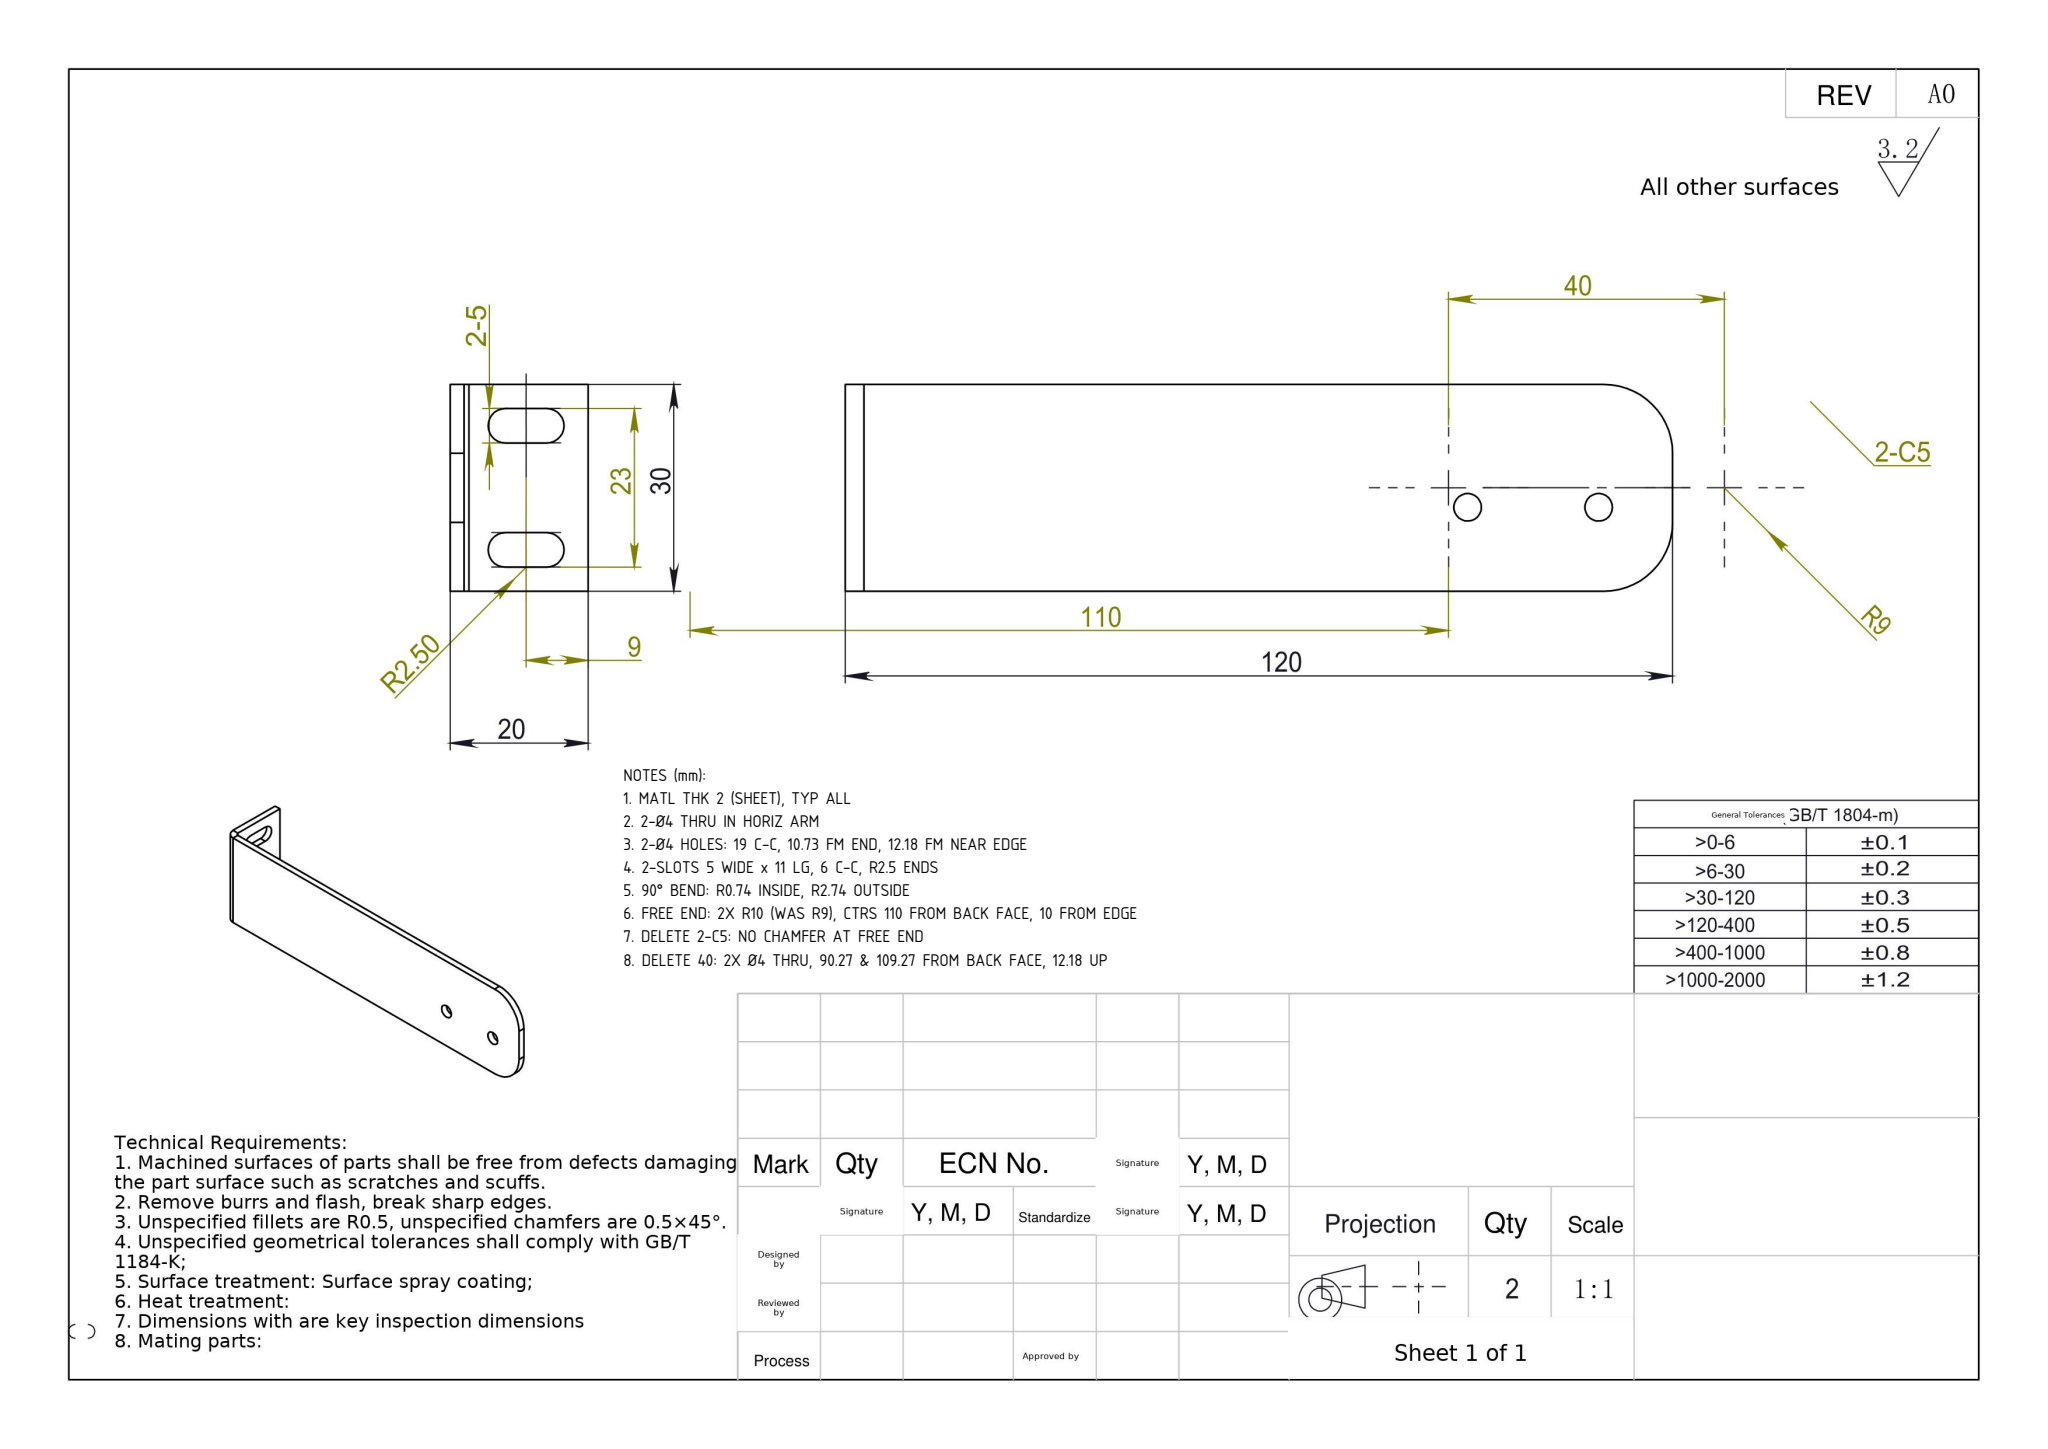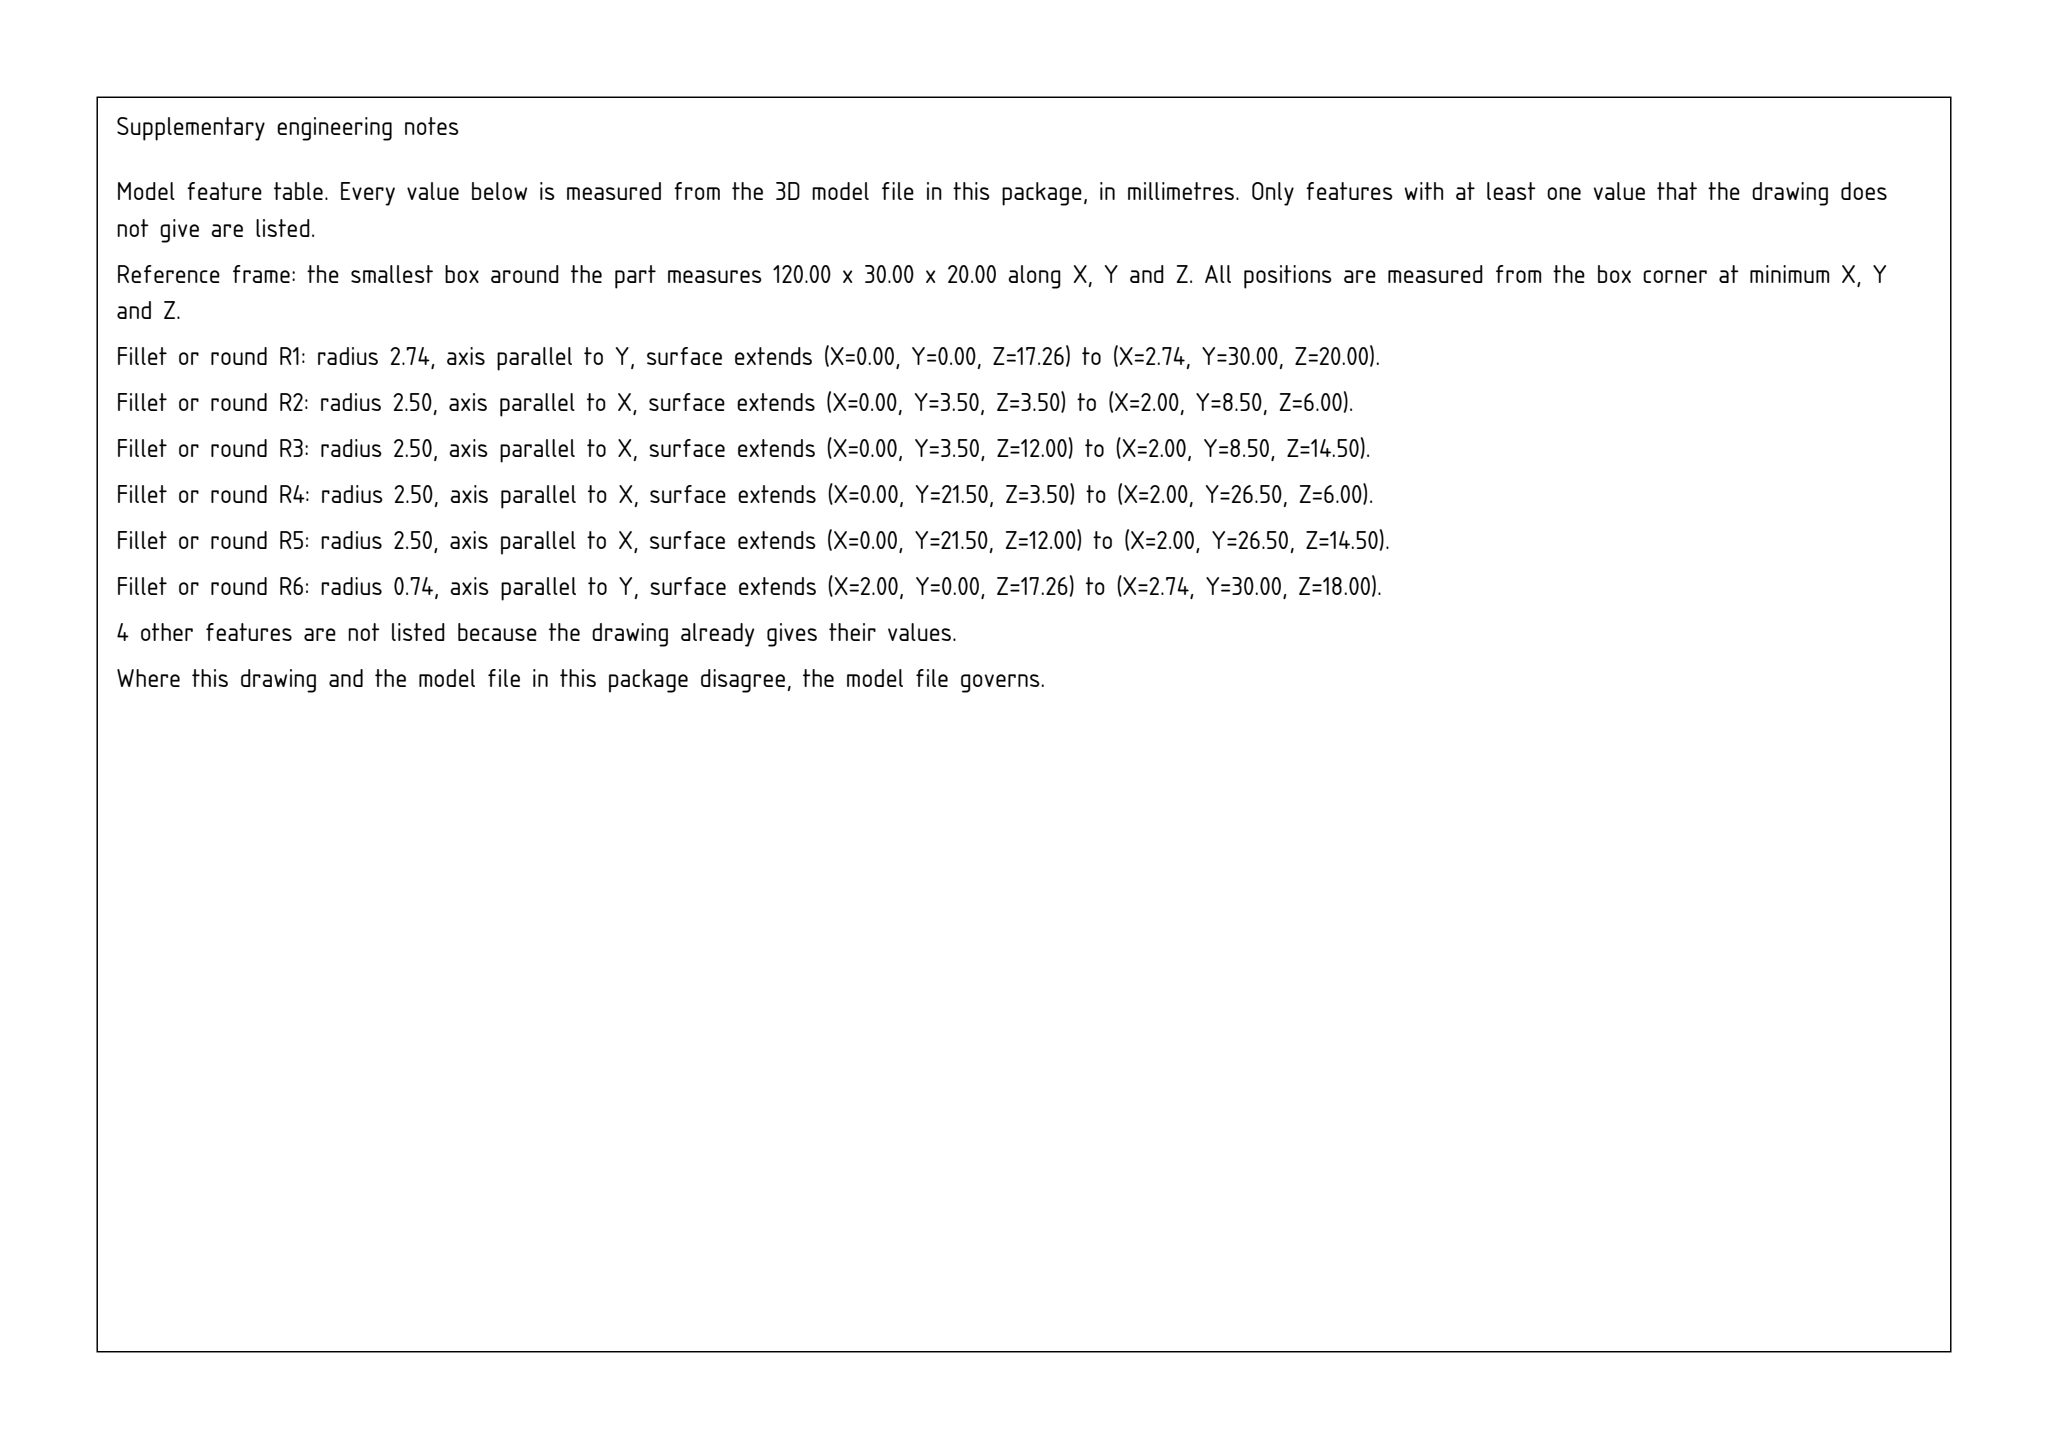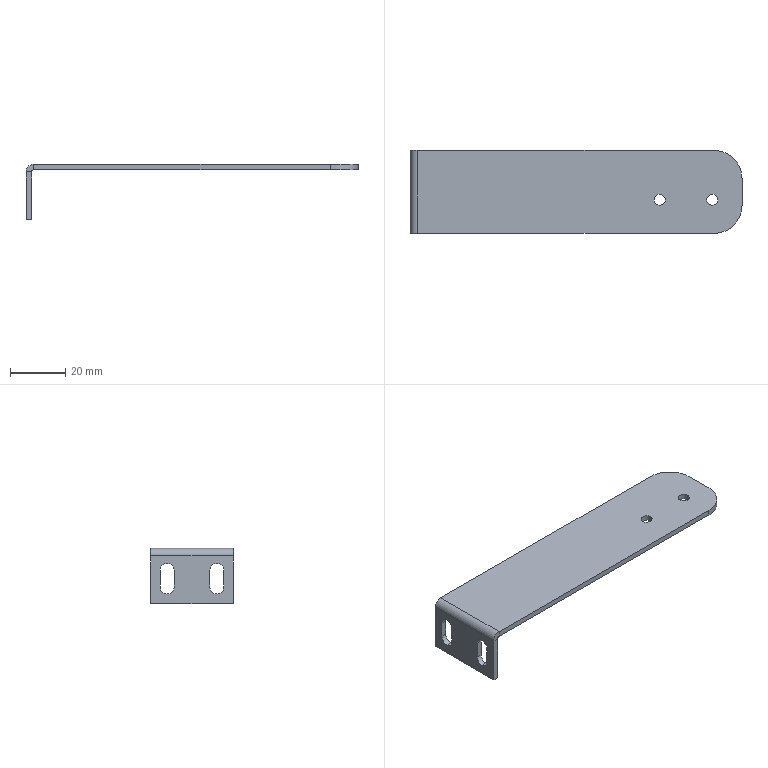Part | SolidWorks | mm | 1 solid | 30 faces | box 120 x 30 x 20 mm | volume 7901 mm3 | plane 16 | cylinder 14 | commonest cylinder face diameters 5 x6 4 x4 20 x2 5.473 x1 1.473 x1
Drawing notes:
MATL THK 2 (SHEET), TYP ALL | from the solid: Parallel faces z=18/z=20 and x=0/x=2 give 2.0 wall
2-Ø4 THRU IN HORIZ ARM | from the solid: cylinders dia 4.0, axis z, length 2 (thru plate), qty 2
2-Ø4 HOLES: 19 C-C, 10.73 FM END, 12.18 FM NEAR EDGE | from the solid: hole axes at x=90.27 & 109.27 (bbox x=0..120), y=12.18 (bbox y=0..30)
2-SLOTS 5 WIDE x 11 LG, 6 C-C, R2.5 ENDS | from the solid: dia 5 cyls, axis x, at z=6 & z=12 for y=6 and y=24
90° BEND: R0.74 INSIDE, R2.74 OUTSIDE | from the solid: cyl dia 1.473 and 5.473, axis y, ctr x=2.74 z=17.26, len 30
FREE END: 2X R10 (WAS R9), CTRS 110 FROM BACK FACE, 10 FROM EDGE | from the solid: cylinders dia 20.0 axis z at [110.0,10.0] and [110.0,20.0], len 2.0 = plate thk; bbox x=120, y=30
DELETE 2-C5: NO CHAMFER AT FREE END | from the solid: cones[] empty, fillet_radii[] empty; free end bounded only by Ø20 (R10) rounds and planes x=120
DELETE 40: 2X Ø4 THRU, 90.27 & 109.27 FROM BACK FACE, 12.18 UP | from the solid: cylinders dia 4.0 axis z at [90.27,12.18] and [109.27,12.18], len 2.0 thru plate; back face = plane x=0